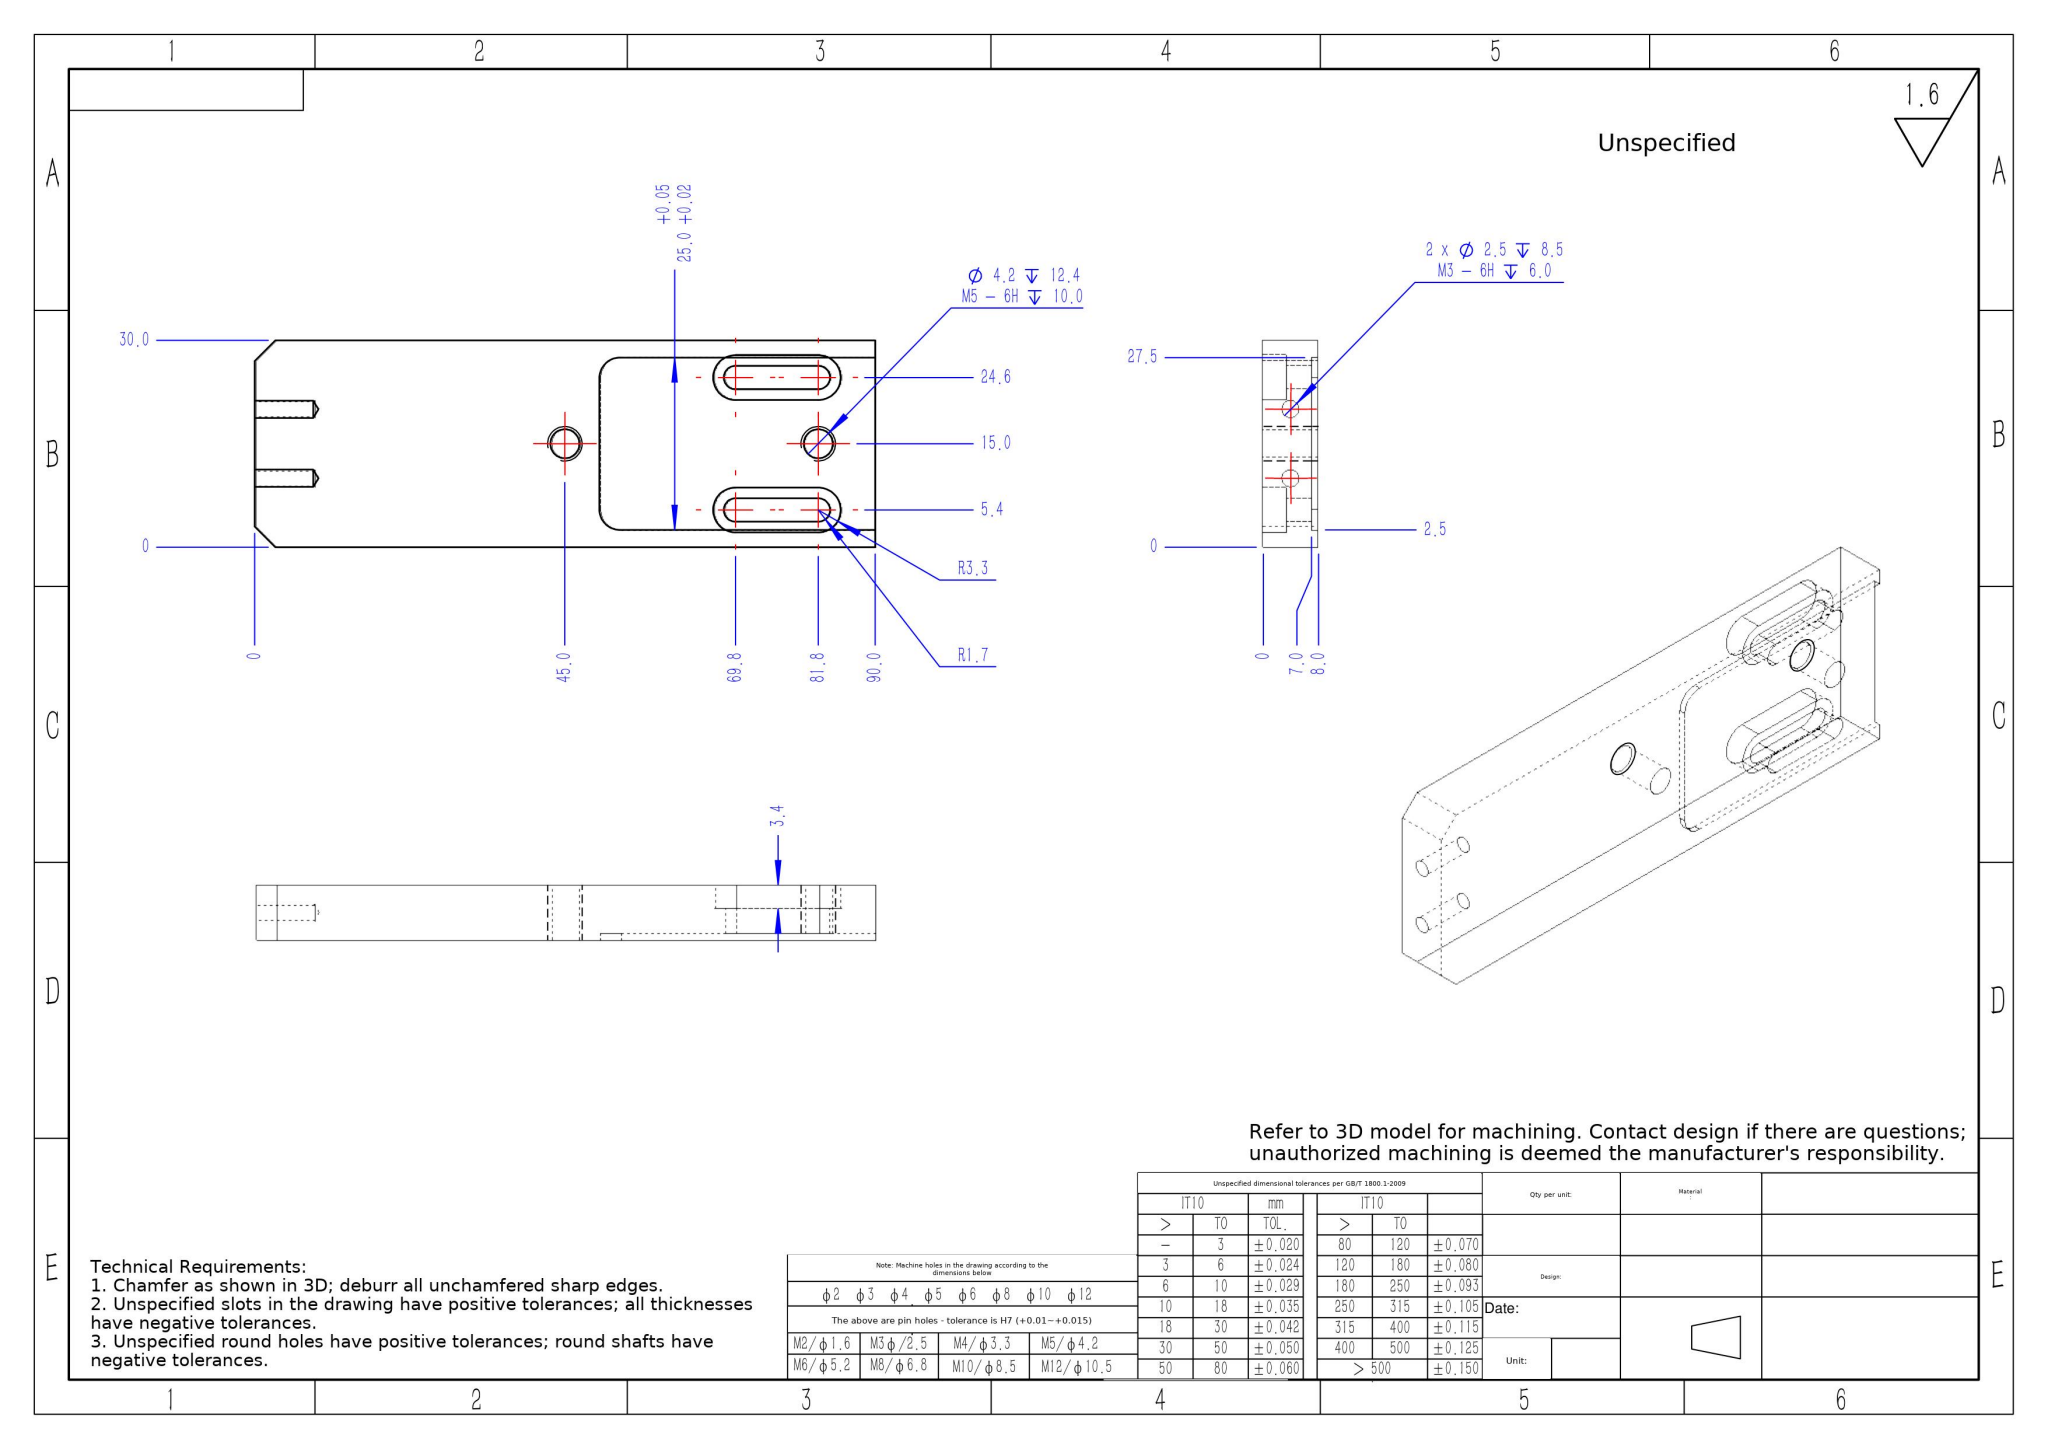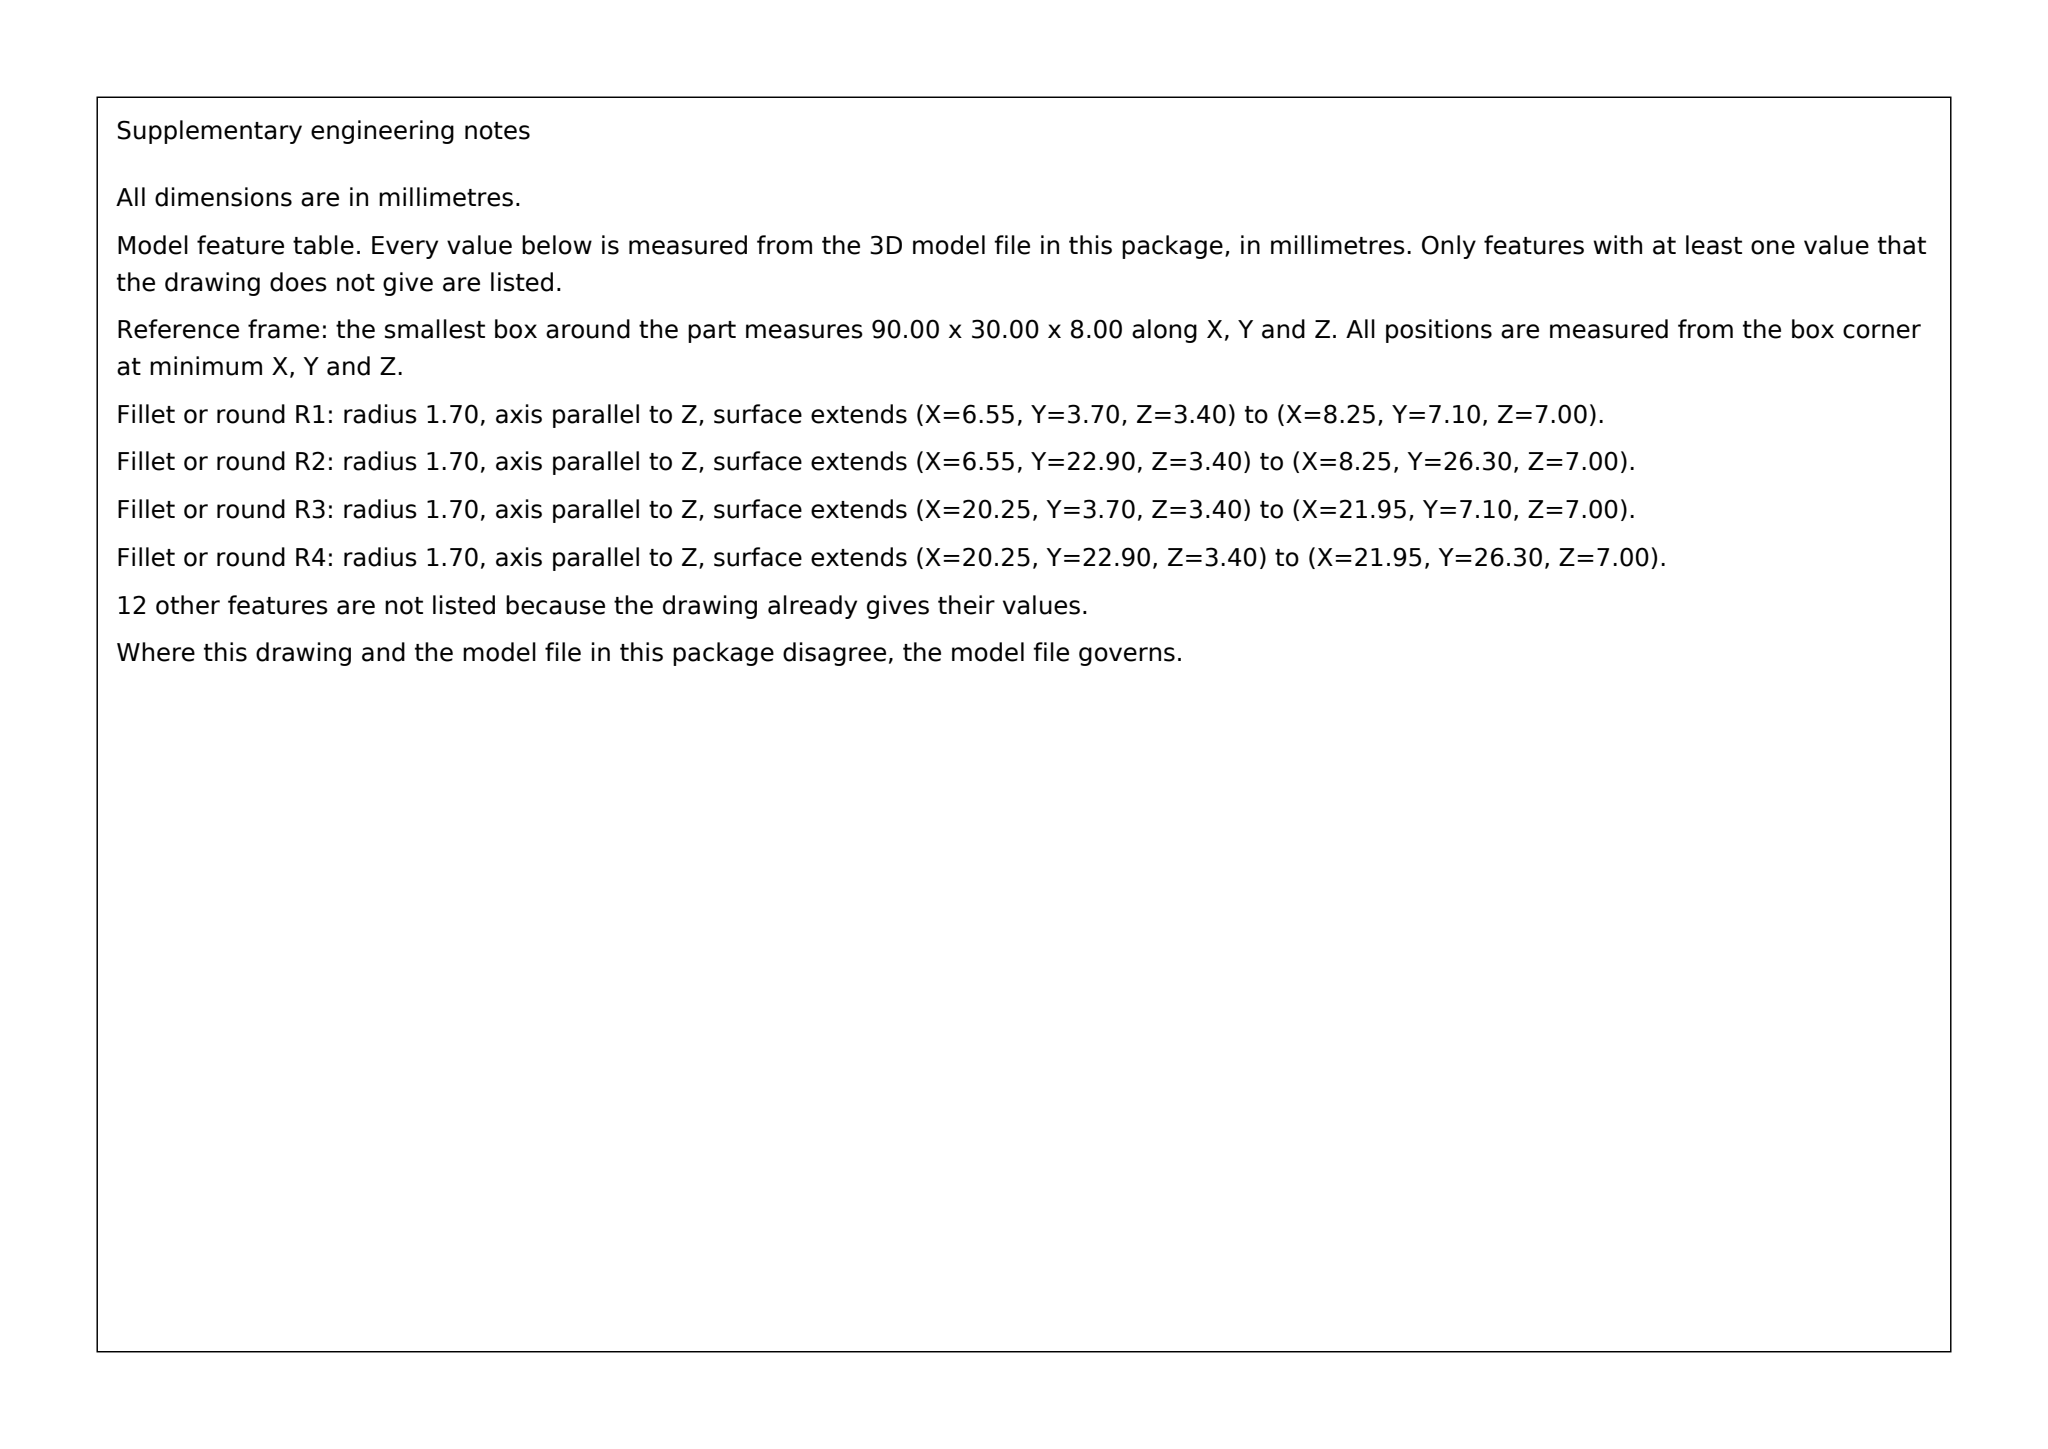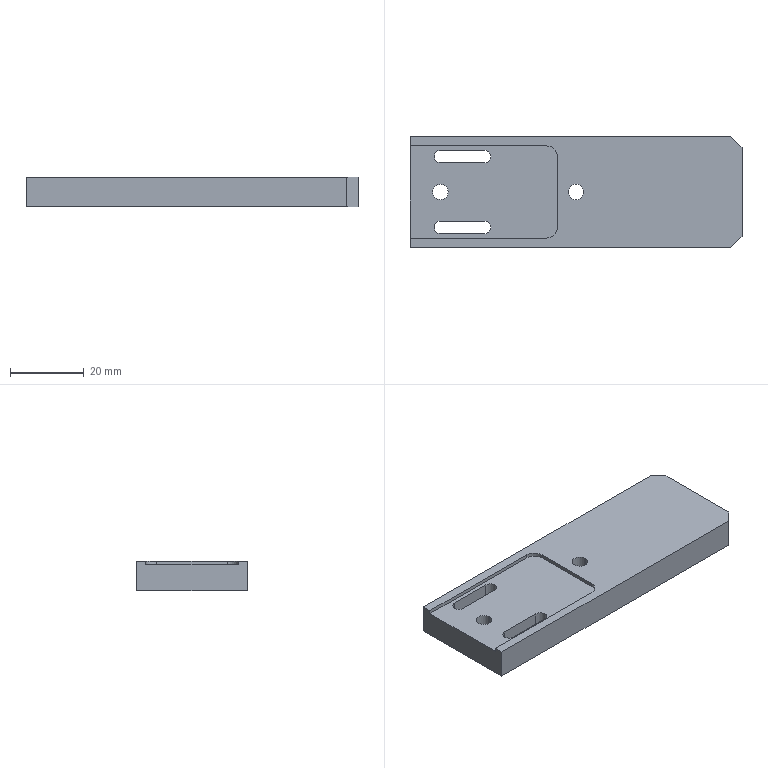Part | SolidWorks | mm | 1 solid | 48 faces | box 90 x 30 x 8 mm | volume 19123 mm3 | cylinder 22 | plane 22 | cone 4 | commonest cylinder face diameters 3.4 x6 6.5 x6 4.2 x4 2.5 x4 6 x2